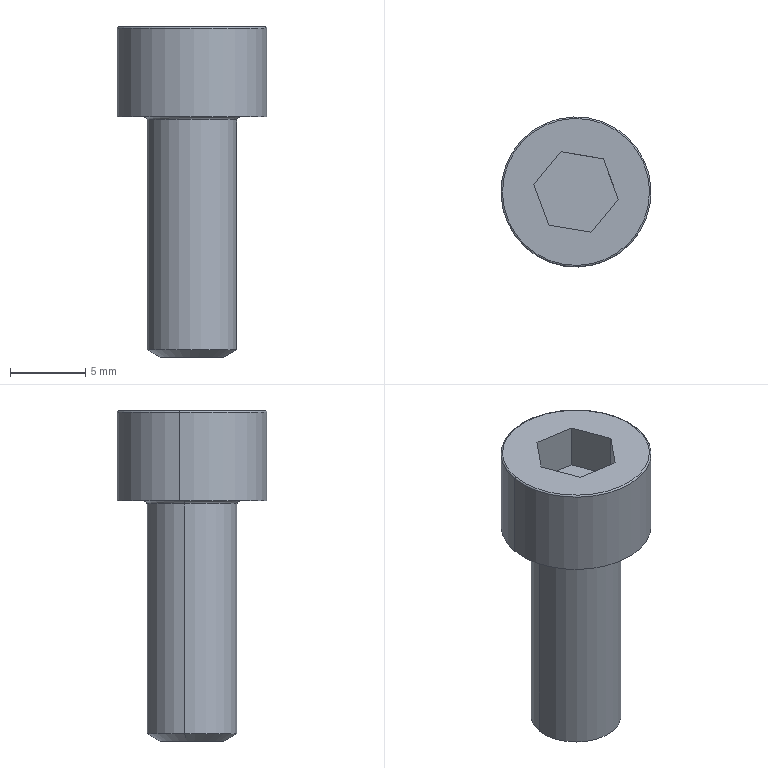Component | SolidWorks | GB_T70.1-2000_SocketHeadCapScrew_M6_16-1 | 1 solid | 20 faces | box 10 x 10 x 22 mm | volume 856 mm3 | plane 10 | torus 4 | cylinder 4 | cone 2 | commonest cylinder face diameters 10 x2 6 x2 | material 8.8 Grade
STEP:
#1=COLOUR_RGB('',0.7922,0.8196,0.9333);
#2=FILL_AREA_STYLE_COLOUR('',#1);
#3=FILL_AREA_STYLE('',(#2));
#4=SURFACE_STYLE_FILL_AREA(#3);
#5=SURFACE_SIDE_STYLE('',(#4));
#6=SURFACE_STYLE_USAGE(.BOTH.,#5);
#7=PRESENTATION_STYLE_ASSIGNMENT((#6));
#8=CARTESIAN_POINT('',(12.001,-2.129,19.252));
#9=VERTEX_POINT('',#8);
#10=CARTESIAN_POINT('',(11.621,-2.064,19.252));
#11=VERTEX_POINT('',#10);
#12=CARTESIAN_POINT('',(11.811,-2.096,19.252));
#13=DIRECTION('',(0.,-0.,1.));
#14=DIRECTION('',(-0.9861,0.1664,0.));
#15=AXIS2_PLACEMENT_3D('',#12,#13,#14);
#16=CIRCLE('',#15,0.1929);
#17=EDGE_CURVE('',#9,#11,#16,.T.);
#18=ORIENTED_EDGE('',*,*,#17,.F.);
#19=CARTESIAN_POINT('',(12.005,-2.129,19.248));
#20=VERTEX_POINT('',#19);
#21=CARTESIAN_POINT('',(12.001,-2.129,19.248));
#22=DIRECTION('',(0.1664,0.9861,-0.));
#23=DIRECTION('',(-0.9861,0.1664,0.));
#24=AXIS2_PLACEMENT_3D('',#21,#22,#23);
#25=CIRCLE('',#24,0.003937);
#26=EDGE_CURVE('',#9,#20,#25,.T.);
#27=ORIENTED_EDGE('',*,*,#26,.T.);
#28=CARTESIAN_POINT('',(11.617,-2.064,19.248));
#29=VERTEX_POINT('',#28);
#30=CARTESIAN_POINT('',(11.811,-2.096,19.248));
#31=DIRECTION('',(-0.,0.,-1.));
#32=DIRECTION('',(-0.9861,0.1664,0.));
#33=AXIS2_PLACEMENT_3D('',#30,#31,#32);
#34=CIRCLE('',#33,0.1969);
#35=EDGE_CURVE('',#29,#20,#34,.T.);
#36=ORIENTED_EDGE('',*,*,#35,.F.);
#37=CARTESIAN_POINT('',(11.621,-2.064,19.248));
#38=DIRECTION('',(-0.1664,-0.9861,0.));
#39=DIRECTION('',(0.9861,-0.1664,0.));
#40=AXIS2_PLACEMENT_3D('',#37,#38,#39);
#41=CIRCLE('',#40,0.003937);
#42=EDGE_CURVE('',#11,#29,#41,.T.);
#43=ORIENTED_EDGE('',*,*,#42,.F.);
#44=EDGE_LOOP('',(#18,#27,#36,#43));
#45=FACE_OUTER_BOUND('',#44,.T.);
#46=CARTESIAN_POINT('',(11.811,-2.096,19.248));
#47=DIRECTION('',(-0.,0.,-1.));
#48=DIRECTION('',(-0.9861,0.1664,0.));
#49=AXIS2_PLACEMENT_3D('',#46,#47,#48);
#50=TOROIDAL_SURFACE('',#49,0.1929,0.003937);
#51=ADVANCED_FACE('',(#45),#50,.T.);
#52=CARTESIAN_POINT('',(11.894,-2.11,18.386));
#53=VERTEX_POINT('',#52);
#54=CARTESIAN_POINT('',(11.728,-2.082,18.386));
#55=VERTEX_POINT('',#54);
#56=CARTESIAN_POINT('',(11.811,-2.096,18.386));
#57=DIRECTION('',(0.,-0.,1.));
#58=DIRECTION('',(0.9861,-0.1664,0.));
#59=AXIS2_PLACEMENT_3D('',#56,#57,#58);
#60=CIRCLE('',#59,0.08402);
#61=EDGE_CURVE('',#53,#55,#60,.T.);
#62=ORIENTED_EDGE('',*,*,#61,.T.);
#63=CARTESIAN_POINT('',(11.695,-2.077,18.406));
#64=VERTEX_POINT('',#63);
#65=CARTESIAN_POINT('',(11.695,-2.077,18.406));
#66=DIRECTION('',(-0.854,0.1441,0.5));
#67=VECTOR('',#66,39.37);
#68=LINE('',#65,#67);
#69=EDGE_CURVE('',#55,#64,#68,.T.);
#70=ORIENTED_EDGE('',*,*,#69,.T.);
#71=CARTESIAN_POINT('',(11.927,-2.116,18.406));
#72=VERTEX_POINT('',#71);
#73=CARTESIAN_POINT('',(11.811,-2.096,18.406));
#74=DIRECTION('',(0.,-0.,1.));
#75=DIRECTION('',(0.9861,-0.1664,0.));
#76=AXIS2_PLACEMENT_3D('',#73,#74,#75);
#77=CIRCLE('',#76,0.1181);
#78=EDGE_CURVE('',#72,#64,#77,.T.);
#79=ORIENTED_EDGE('',*,*,#78,.F.);
#80=CARTESIAN_POINT('',(11.927,-2.116,18.406));
#81=DIRECTION('',(0.854,-0.1441,0.5));
#82=VECTOR('',#81,39.37);
#83=LINE('',#80,#82);
#84=EDGE_CURVE('',#53,#72,#83,.T.);
#85=ORIENTED_EDGE('',*,*,#84,.F.);
#86=EDGE_LOOP('',(#62,#70,#79,#85));
#87=FACE_OUTER_BOUND('',#86,.T.);
#88=CARTESIAN_POINT('',(11.811,-2.096,18.406));
#89=DIRECTION('',(0.,-0.,1.));
#90=DIRECTION('',(0.9861,-0.1664,0.));
#91=AXIS2_PLACEMENT_3D('',#88,#89,#90);
#92=CONICAL_SURFACE('',#91,0.1181,1.047);
#93=ADVANCED_FACE('',(#87),#92,.T.);
#94=CARTESIAN_POINT('',(11.687,-2.075,19.016));
#95=VERTEX_POINT('',#94);
#96=CARTESIAN_POINT('',(11.935,-2.117,19.016));
#97=VERTEX_POINT('',#96);
#98=CARTESIAN_POINT('',(11.811,-2.096,19.016));
#99=DIRECTION('',(0.,-0.,1.));
#100=DIRECTION('',(0.9861,-0.1664,0.));
#101=AXIS2_PLACEMENT_3D('',#98,#99,#100);
#102=CIRCLE('',#101,0.126);
#103=EDGE_CURVE('',#95,#97,#102,.T.);
#104=ORIENTED_EDGE('',*,*,#103,.F.);
#105=CARTESIAN_POINT('',(11.695,-2.077,19.008));
#106=VERTEX_POINT('',#105);
#107=CARTESIAN_POINT('',(11.687,-2.075,19.008));
#108=DIRECTION('',(0.1664,0.9861,-0.));
#109=DIRECTION('',(-0.9861,0.1664,0.));
#110=AXIS2_PLACEMENT_3D('',#107,#108,#109);
#111=CIRCLE('',#110,0.007874);
#112=EDGE_CURVE('',#95,#106,#111,.T.);
#113=ORIENTED_EDGE('',*,*,#112,.T.);
#114=CARTESIAN_POINT('',(11.927,-2.116,19.008));
#115=VERTEX_POINT('',#114);
#116=CARTESIAN_POINT('',(11.811,-2.096,19.008));
#117=DIRECTION('',(0.,-0.,1.));
#118=DIRECTION('',(0.9861,-0.1664,0.));
#119=AXIS2_PLACEMENT_3D('',#116,#117,#118);
#120=CIRCLE('',#119,0.1181);
#121=EDGE_CURVE('',#106,#115,#120,.T.);
#122=ORIENTED_EDGE('',*,*,#121,.T.);
#123=CARTESIAN_POINT('',(11.935,-2.117,19.008));
#124=DIRECTION('',(-0.1664,-0.9861,0.));
#125=DIRECTION('',(0.9861,-0.1664,0.));
#126=AXIS2_PLACEMENT_3D('',#123,#124,#125);
#127=CIRCLE('',#126,0.007874);
#128=EDGE_CURVE('',#97,#115,#127,.T.);
#129=ORIENTED_EDGE('',*,*,#128,.F.);
#130=EDGE_LOOP('',(#104,#113,#122,#129));
#131=FACE_OUTER_BOUND('',#130,.T.);
#132=CARTESIAN_POINT('',(11.811,-2.096,19.008));
#133=DIRECTION('',(0.,-0.,1.));
#134=DIRECTION('',(0.9861,-0.1664,-0.));
#135=AXIS2_PLACEMENT_3D('',#132,#133,#134);
#136=TOROIDAL_SURFACE('',#135,0.126,0.007874);
#137=ADVANCED_FACE('',(#131),#136,.F.);
#138=CARTESIAN_POINT('',(12.005,-2.129,19.016));
#139=VERTEX_POINT('',#138);
#140=CARTESIAN_POINT('',(11.617,-2.064,19.016));
#141=VERTEX_POINT('',#140);
#142=CARTESIAN_POINT('',(11.811,-2.096,19.016));
#143=DIRECTION('',(0.,-0.,1.));
#144=DIRECTION('',(0.9861,-0.1664,0.));
#145=AXIS2_PLACEMENT_3D('',#142,#143,#144);
#146=CIRCLE('',#145,0.1969);
#147=EDGE_CURVE('',#139,#141,#146,.T.);
#148=ORIENTED_EDGE('',*,*,#147,.T.);
#149=CARTESIAN_POINT('',(11.617,-2.064,19.252));
#150=DIRECTION('',(0.,-0.,1.));
#151=VECTOR('',#150,39.37);
#152=LINE('',#149,#151);
#153=EDGE_CURVE('',#141,#29,#152,.T.);
#154=ORIENTED_EDGE('',*,*,#153,.T.);
#155=ORIENTED_EDGE('',*,*,#35,.T.);
#156=CARTESIAN_POINT('',(12.005,-2.129,19.252));
#157=DIRECTION('',(0.,-0.,1.));
#158=VECTOR('',#157,39.37);
#159=LINE('',#156,#158);
#160=EDGE_CURVE('',#139,#20,#159,.T.);
#161=ORIENTED_EDGE('',*,*,#160,.F.);
#162=EDGE_LOOP('',(#148,#154,#155,#161));
#163=FACE_OUTER_BOUND('',#162,.T.);
#164=CARTESIAN_POINT('',(11.811,-2.096,19.252));
#165=DIRECTION('',(0.,-0.,1.));
#166=DIRECTION('',(0.9861,-0.1664,0.));
#167=AXIS2_PLACEMENT_3D('',#164,#165,#166);
#168=CYLINDRICAL_SURFACE('',#167,0.1969);
#169=ADVANCED_FACE('',(#163),#168,.T.);
#170=ORIENTED_EDGE('',*,*,#78,.T.);
#171=CARTESIAN_POINT('',(11.695,-2.077,19.252));
#172=DIRECTION('',(0.,-0.,1.));
#173=VECTOR('',#172,39.37);
#174=LINE('',#171,#173);
#175=EDGE_CURVE('',#64,#106,#174,.T.);
#176=ORIENTED_EDGE('',*,*,#175,.T.);
#177=CARTESIAN_POINT('',(11.811,-2.096,19.008));
#178=DIRECTION('',(0.,-0.,1.));
#179=DIRECTION('',(0.9861,-0.1664,0.));
#180=AXIS2_PLACEMENT_3D('',#177,#178,#179);
#181=CIRCLE('',#180,0.1181);
#182=EDGE_CURVE('',#115,#106,#181,.T.);
#183=ORIENTED_EDGE('',*,*,#182,.F.);
#184=CARTESIAN_POINT('',(11.927,-2.116,19.252));
#185=DIRECTION('',(0.,-0.,1.));
#186=VECTOR('',#185,39.37);
#187=LINE('',#184,#186);
#188=EDGE_CURVE('',#72,#115,#187,.T.);
#189=ORIENTED_EDGE('',*,*,#188,.F.);
#190=EDGE_LOOP('',(#170,#176,#183,#189));
#191=FACE_OUTER_BOUND('',#190,.T.);
#192=CARTESIAN_POINT('',(11.811,-2.096,19.252));
#193=DIRECTION('',(0.,-0.,1.));
#194=DIRECTION('',(0.9861,-0.1664,0.));
#195=AXIS2_PLACEMENT_3D('',#192,#193,#194);
#196=CYLINDRICAL_SURFACE('',#195,0.1181);
#197=ADVANCED_FACE('',(#191),#196,.T.);
#198=ORIENTED_EDGE('',*,*,#175,.F.);
#199=CARTESIAN_POINT('',(11.811,-2.096,18.406));
#200=DIRECTION('',(0.,-0.,1.));
#201=DIRECTION('',(0.9861,-0.1664,0.));
#202=AXIS2_PLACEMENT_3D('',#199,#200,#201);
#203=CIRCLE('',#202,0.1181);
#204=EDGE_CURVE('',#64,#72,#203,.T.);
#205=ORIENTED_EDGE('',*,*,#204,.T.);
#206=ORIENTED_EDGE('',*,*,#188,.T.);
#207=ORIENTED_EDGE('',*,*,#121,.F.);
#208=EDGE_LOOP('',(#198,#205,#206,#207));
#209=FACE_OUTER_BOUND('',#208,.T.);
#210=CARTESIAN_POINT('',(11.811,-2.096,19.252));
#211=DIRECTION('',(0.,-0.,1.));
#212=DIRECTION('',(0.9861,-0.1664,0.));
#213=AXIS2_PLACEMENT_3D('',#210,#211,#212);
#214=CYLINDRICAL_SURFACE('',#213,0.1181);
#215=ADVANCED_FACE('',(#209),#214,.T.);
#216=CARTESIAN_POINT('',(11.811,-2.096,19.252));
#217=DIRECTION('',(0.,-0.,1.));
#218=DIRECTION('',(-0.9861,0.1664,0.));
#219=AXIS2_PLACEMENT_3D('',#216,#217,#218);
#220=CIRCLE('',#219,0.1929);
#221=EDGE_CURVE('',#11,#9,#220,.T.);
#222=ORIENTED_EDGE('',*,*,#221,.T.);
#223=ORIENTED_EDGE('',*,*,#17,.T.);
#224=EDGE_LOOP('',(#222,#223));
#225=FACE_OUTER_BOUND('',#224,.T.);
#226=CARTESIAN_POINT('',(11.922,-2.115,19.252));
#227=VERTEX_POINT('',#226);
#228=CARTESIAN_POINT('',(11.883,-2.01,19.252));
#229=VERTEX_POINT('',#228);
#230=CARTESIAN_POINT('',(11.922,-2.115,19.252));
#231=DIRECTION('',(-0.3489,0.9371,0.));
#232=VECTOR('',#231,39.37);
#233=LINE('',#230,#232);
#234=EDGE_CURVE('',#227,#229,#233,.T.);
#235=ORIENTED_EDGE('',*,*,#234,.F.);
#236=CARTESIAN_POINT('',(11.85,-2.202,19.252));
#237=VERTEX_POINT('',#236);
#238=CARTESIAN_POINT('',(11.85,-2.202,19.252));
#239=DIRECTION('',(0.6371,0.7708,-0.));
#240=VECTOR('',#239,39.37);
#241=LINE('',#238,#240);
#242=EDGE_CURVE('',#237,#227,#241,.T.);
#243=ORIENTED_EDGE('',*,*,#242,.F.);
#244=CARTESIAN_POINT('',(11.739,-2.183,19.252));
#245=VERTEX_POINT('',#244);
#246=CARTESIAN_POINT('',(11.739,-2.183,19.252));
#247=DIRECTION('',(0.9861,-0.1664,-0.));
#248=VECTOR('',#247,39.37);
#249=LINE('',#246,#248);
#250=EDGE_CURVE('',#245,#237,#249,.T.);
#251=ORIENTED_EDGE('',*,*,#250,.F.);
#252=CARTESIAN_POINT('',(11.7,-2.078,19.252));
#253=VERTEX_POINT('',#252);
#254=CARTESIAN_POINT('',(11.7,-2.078,19.252));
#255=DIRECTION('',(0.3489,-0.9371,-0.));
#256=VECTOR('',#255,39.37);
#257=LINE('',#254,#256);
#258=EDGE_CURVE('',#253,#245,#257,.T.);
#259=ORIENTED_EDGE('',*,*,#258,.F.);
#260=CARTESIAN_POINT('',(11.772,-1.991,19.252));
#261=VERTEX_POINT('',#260);
#262=CARTESIAN_POINT('',(11.772,-1.991,19.252));
#263=DIRECTION('',(-0.6371,-0.7708,0.));
#264=VECTOR('',#263,39.37);
#265=LINE('',#262,#264);
#266=EDGE_CURVE('',#261,#253,#265,.T.);
#267=ORIENTED_EDGE('',*,*,#266,.F.);
#268=CARTESIAN_POINT('',(11.883,-2.01,19.252));
#269=DIRECTION('',(-0.9861,0.1664,0.));
#270=VECTOR('',#269,39.37);
#271=LINE('',#268,#270);
#272=EDGE_CURVE('',#229,#261,#271,.T.);
#273=ORIENTED_EDGE('',*,*,#272,.F.);
#274=EDGE_LOOP('',(#235,#243,#251,#259,#267,#273));
#275=FACE_BOUND('',#274,.T.);
#276=CARTESIAN_POINT('',(11.811,-2.096,19.252));
#277=DIRECTION('',(-0.,0.,-1.));
#278=DIRECTION('',(-0.9861,0.1664,0.));
#279=AXIS2_PLACEMENT_3D('',#276,#277,#278);
#280=PLANE('',#279);
#281=ADVANCED_FACE('',(#225,#275),#280,.F.);
#282=ORIENTED_EDGE('',*,*,#153,.F.);
#283=CARTESIAN_POINT('',(11.811,-2.096,19.016));
#284=DIRECTION('',(0.,-0.,1.));
#285=DIRECTION('',(0.9861,-0.1664,0.));
#286=AXIS2_PLACEMENT_3D('',#283,#284,#285);
#287=CIRCLE('',#286,0.1969);
#288=EDGE_CURVE('',#141,#139,#287,.T.);
#289=ORIENTED_EDGE('',*,*,#288,.T.);
#290=ORIENTED_EDGE('',*,*,#160,.T.);
#291=CARTESIAN_POINT('',(11.811,-2.096,19.248));
#292=DIRECTION('',(-0.,0.,-1.));
#293=DIRECTION('',(-0.9861,0.1664,0.));
#294=AXIS2_PLACEMENT_3D('',#291,#292,#293);
#295=CIRCLE('',#294,0.1969);
#296=EDGE_CURVE('',#20,#29,#295,.T.);
#297=ORIENTED_EDGE('',*,*,#296,.T.);
#298=EDGE_LOOP('',(#282,#289,#290,#297));
#299=FACE_OUTER_BOUND('',#298,.T.);
#300=CARTESIAN_POINT('',(11.811,-2.096,19.252));
#301=DIRECTION('',(0.,-0.,1.));
#302=DIRECTION('',(0.9861,-0.1664,0.));
#303=AXIS2_PLACEMENT_3D('',#300,#301,#302);
#304=CYLINDRICAL_SURFACE('',#303,0.1969);
#305=ADVANCED_FACE('',(#299),#304,.T.);
#306=ORIENTED_EDGE('',*,*,#147,.F.);
#307=ORIENTED_EDGE('',*,*,#288,.F.);
#308=EDGE_LOOP('',(#306,#307));
#309=FACE_OUTER_BOUND('',#308,.T.);
#310=CARTESIAN_POINT('',(11.811,-2.096,19.016));
#311=DIRECTION('',(0.,-0.,1.));
#312=DIRECTION('',(0.9861,-0.1664,0.));
#313=AXIS2_PLACEMENT_3D('',#310,#311,#312);
#314=CIRCLE('',#313,0.126);
#315=EDGE_CURVE('',#97,#95,#314,.T.);
#316=ORIENTED_EDGE('',*,*,#315,.T.);
#317=ORIENTED_EDGE('',*,*,#103,.T.);
#318=EDGE_LOOP('',(#316,#317));
#319=FACE_BOUND('',#318,.T.);
#320=CARTESIAN_POINT('',(11.844,-1.902,19.016));
#321=DIRECTION('',(0.,-0.,1.));
#322=DIRECTION('',(0.9861,-0.1664,-0.));
#323=AXIS2_PLACEMENT_3D('',#320,#321,#322);
#324=PLANE('',#323);
#325=ADVANCED_FACE('',(#309,#319),#324,.F.);
#326=ORIENTED_EDGE('',*,*,#112,.F.);
#327=ORIENTED_EDGE('',*,*,#315,.F.);
#328=ORIENTED_EDGE('',*,*,#128,.T.);
#329=ORIENTED_EDGE('',*,*,#182,.T.);
#330=EDGE_LOOP('',(#326,#327,#328,#329));
#331=FACE_OUTER_BOUND('',#330,.T.);
#332=CARTESIAN_POINT('',(11.811,-2.096,19.008));
#333=DIRECTION('',(0.,-0.,1.));
#334=DIRECTION('',(0.9861,-0.1664,-0.));
#335=AXIS2_PLACEMENT_3D('',#332,#333,#334);
#336=TOROIDAL_SURFACE('',#335,0.126,0.007874);
#337=ADVANCED_FACE('',(#331),#336,.F.);
#338=ORIENTED_EDGE('',*,*,#242,.T.);
#339=CARTESIAN_POINT('',(11.922,-2.115,19.134));
#340=VERTEX_POINT('',#339);
#341=CARTESIAN_POINT('',(11.922,-2.115,19.134));
#342=DIRECTION('',(0.,-0.,1.));
#343=VECTOR('',#342,39.37);
#344=LINE('',#341,#343);
#345=EDGE_CURVE('',#340,#227,#344,.T.);
#346=ORIENTED_EDGE('',*,*,#345,.F.);
#347=CARTESIAN_POINT('',(11.85,-2.202,19.134));
#348=VERTEX_POINT('',#347);
#349=CARTESIAN_POINT('',(11.85,-2.202,19.134));
#350=DIRECTION('',(0.6371,0.7708,-0.));
#351=VECTOR('',#350,39.37);
#352=LINE('',#349,#351);
#353=EDGE_CURVE('',#348,#340,#352,.T.);
#354=ORIENTED_EDGE('',*,*,#353,.F.);
#355=CARTESIAN_POINT('',(11.85,-2.202,19.134));
#356=DIRECTION('',(0.,-0.,1.));
#357=VECTOR('',#356,39.37);
#358=LINE('',#355,#357);
#359=EDGE_CURVE('',#348,#237,#358,.T.);
#360=ORIENTED_EDGE('',*,*,#359,.T.);
#361=EDGE_LOOP('',(#338,#346,#354,#360));
#362=FACE_OUTER_BOUND('',#361,.T.);
#363=CARTESIAN_POINT('',(11.85,-2.202,19.134));
#364=DIRECTION('',(0.7708,-0.6371,-0.));
#365=DIRECTION('',(-0.6371,-0.7708,0.));
#366=AXIS2_PLACEMENT_3D('',#363,#364,#365);
#367=PLANE('',#366);
#368=ADVANCED_FACE('',(#362),#367,.F.);
#369=ORIENTED_EDGE('',*,*,#250,.T.);
#370=ORIENTED_EDGE('',*,*,#359,.F.);
#371=CARTESIAN_POINT('',(11.739,-2.183,19.134));
#372=VERTEX_POINT('',#371);
#373=CARTESIAN_POINT('',(11.739,-2.183,19.134));
#374=DIRECTION('',(0.9861,-0.1664,-0.));
#375=VECTOR('',#374,39.37);
#376=LINE('',#373,#375);
#377=EDGE_CURVE('',#372,#348,#376,.T.);
#378=ORIENTED_EDGE('',*,*,#377,.F.);
#379=CARTESIAN_POINT('',(11.739,-2.183,19.134));
#380=DIRECTION('',(0.,-0.,1.));
#381=VECTOR('',#380,39.37);
#382=LINE('',#379,#381);
#383=EDGE_CURVE('',#372,#245,#382,.T.);
#384=ORIENTED_EDGE('',*,*,#383,.T.);
#385=EDGE_LOOP('',(#369,#370,#378,#384));
#386=FACE_OUTER_BOUND('',#385,.T.);
#387=CARTESIAN_POINT('',(11.739,-2.183,19.134));
#388=DIRECTION('',(-0.1664,-0.9861,0.));
#389=DIRECTION('',(-0.9861,0.1664,0.));
#390=AXIS2_PLACEMENT_3D('',#387,#388,#389);
#391=PLANE('',#390);
#392=ADVANCED_FACE('',(#386),#391,.F.);
#393=ORIENTED_EDGE('',*,*,#258,.T.);
#394=ORIENTED_EDGE('',*,*,#383,.F.);
#395=CARTESIAN_POINT('',(11.7,-2.078,19.134));
#396=VERTEX_POINT('',#395);
#397=CARTESIAN_POINT('',(11.7,-2.078,19.134));
#398=DIRECTION('',(0.3489,-0.9371,-0.));
#399=VECTOR('',#398,39.37);
#400=LINE('',#397,#399);
#401=EDGE_CURVE('',#396,#372,#400,.T.);
#402=ORIENTED_EDGE('',*,*,#401,.F.);
#403=CARTESIAN_POINT('',(11.7,-2.078,19.134));
#404=DIRECTION('',(0.,-0.,1.));
#405=VECTOR('',#404,39.37);
#406=LINE('',#403,#405);
#407=EDGE_CURVE('',#396,#253,#406,.T.);
#408=ORIENTED_EDGE('',*,*,#407,.T.);
#409=EDGE_LOOP('',(#393,#394,#402,#408));
#410=FACE_OUTER_BOUND('',#409,.T.);
#411=CARTESIAN_POINT('',(11.7,-2.078,19.134));
#412=DIRECTION('',(-0.9371,-0.3489,0.));
#413=DIRECTION('',(-0.3489,0.9371,0.));
#414=AXIS2_PLACEMENT_3D('',#411,#412,#413);
#415=PLANE('',#414);
#416=ADVANCED_FACE('',(#410),#415,.F.);
#417=ORIENTED_EDGE('',*,*,#266,.T.);
#418=ORIENTED_EDGE('',*,*,#407,.F.);
#419=CARTESIAN_POINT('',(11.772,-1.991,19.134));
#420=VERTEX_POINT('',#419);
#421=CARTESIAN_POINT('',(11.772,-1.991,19.134));
#422=DIRECTION('',(-0.6371,-0.7708,0.));
#423=VECTOR('',#422,39.37);
#424=LINE('',#421,#423);
#425=EDGE_CURVE('',#420,#396,#424,.T.);
#426=ORIENTED_EDGE('',*,*,#425,.F.);
#427=CARTESIAN_POINT('',(11.772,-1.991,19.134));
#428=DIRECTION('',(0.,-0.,1.));
#429=VECTOR('',#428,39.37);
#430=LINE('',#427,#429);
#431=EDGE_CURVE('',#420,#261,#430,.T.);
#432=ORIENTED_EDGE('',*,*,#431,.T.);
#433=EDGE_LOOP('',(#417,#418,#426,#432));
#434=FACE_OUTER_BOUND('',#433,.T.);
#435=CARTESIAN_POINT('',(11.772,-1.991,19.134));
#436=DIRECTION('',(-0.7708,0.6371,0.));
#437=DIRECTION('',(0.6371,0.7708,-0.));
#438=AXIS2_PLACEMENT_3D('',#435,#436,#437);
#439=PLANE('',#438);
#440=ADVANCED_FACE('',(#434),#439,.F.);
#441=ORIENTED_EDGE('',*,*,#272,.T.);
#442=ORIENTED_EDGE('',*,*,#431,.F.);
#443=CARTESIAN_POINT('',(11.883,-2.01,19.134));
#444=VERTEX_POINT('',#443);
#445=CARTESIAN_POINT('',(11.883,-2.01,19.134));
#446=DIRECTION('',(-0.9861,0.1664,0.));
#447=VECTOR('',#446,39.37);
#448=LINE('',#445,#447);
#449=EDGE_CURVE('',#444,#420,#448,.T.);
#450=ORIENTED_EDGE('',*,*,#449,.F.);
#451=CARTESIAN_POINT('',(11.883,-2.01,19.134));
#452=DIRECTION('',(0.,-0.,1.));
#453=VECTOR('',#452,39.37);
#454=LINE('',#451,#453);
#455=EDGE_CURVE('',#444,#229,#454,.T.);
#456=ORIENTED_EDGE('',*,*,#455,.T.);
#457=EDGE_LOOP('',(#441,#442,#450,#456));
#458=FACE_OUTER_BOUND('',#457,.T.);
#459=CARTESIAN_POINT('',(11.883,-2.01,19.134));
#460=DIRECTION('',(0.1664,0.9861,-0.));
#461=DIRECTION('',(0.9861,-0.1664,-0.));
#462=AXIS2_PLACEMENT_3D('',#459,#460,#461);
#463=PLANE('',#462);
#464=ADVANCED_FACE('',(#458),#463,.F.);
#465=ORIENTED_EDGE('',*,*,#234,.T.);
#466=ORIENTED_EDGE('',*,*,#455,.F.);
#467=CARTESIAN_POINT('',(11.922,-2.115,19.134));
#468=DIRECTION('',(-0.3489,0.9371,0.));
#469=VECTOR('',#468,39.37);
#470=LINE('',#467,#469);
#471=EDGE_CURVE('',#340,#444,#470,.T.);
#472=ORIENTED_EDGE('',*,*,#471,.F.);
#473=ORIENTED_EDGE('',*,*,#345,.T.);
#474=EDGE_LOOP('',(#465,#466,#472,#473));
#475=FACE_OUTER_BOUND('',#474,.T.);
#476=CARTESIAN_POINT('',(11.922,-2.115,19.134));
#477=DIRECTION('',(0.9371,0.3489,-0.));
#478=DIRECTION('',(0.3489,-0.9371,-0.));
#479=AXIS2_PLACEMENT_3D('',#476,#477,#478);
#480=PLANE('',#479);
#481=ADVANCED_FACE('',(#475),#480,.F.);
#482=ORIENTED_EDGE('',*,*,#353,.T.);
#483=ORIENTED_EDGE('',*,*,#471,.T.);
#484=ORIENTED_EDGE('',*,*,#449,.T.);
#485=ORIENTED_EDGE('',*,*,#425,.T.);
#486=ORIENTED_EDGE('',*,*,#401,.T.);
#487=ORIENTED_EDGE('',*,*,#377,.T.);
#488=EDGE_LOOP('',(#482,#483,#484,#485,#486,#487));
#489=FACE_OUTER_BOUND('',#488,.T.);
#490=CARTESIAN_POINT('',(11.85,-2.202,19.134));
#491=DIRECTION('',(-0.,0.,-1.));
#492=DIRECTION('',(-0.9861,0.1664,0.));
#493=AXIS2_PLACEMENT_3D('',#490,#491,#492);
#494=PLANE('',#493);
#495=ADVANCED_FACE('',(#489),#494,.F.);
#496=ORIENTED_EDGE('',*,*,#69,.F.);
#497=CARTESIAN_POINT('',(11.811,-2.096,18.386));
#498=DIRECTION('',(0.,-0.,1.));
#499=DIRECTION('',(0.9861,-0.1664,0.));
#500=AXIS2_PLACEMENT_3D('',#497,#498,#499);
#501=CIRCLE('',#500,0.08402);
#502=EDGE_CURVE('',#55,#53,#501,.T.);
#503=ORIENTED_EDGE('',*,*,#502,.T.);
#504=ORIENTED_EDGE('',*,*,#84,.T.);
#505=ORIENTED_EDGE('',*,*,#204,.F.);
#506=EDGE_LOOP('',(#496,#503,#504,#505));
#507=FACE_OUTER_BOUND('',#506,.T.);
#508=CARTESIAN_POINT('',(11.811,-2.096,18.406));
#509=DIRECTION('',(0.,-0.,1.));
#510=DIRECTION('',(0.9861,-0.1664,0.));
#511=AXIS2_PLACEMENT_3D('',#508,#509,#510);
#512=CONICAL_SURFACE('',#511,0.1181,1.047);
#513=ADVANCED_FACE('',(#507),#512,.T.);
#514=ORIENTED_EDGE('',*,*,#61,.F.);
#515=ORIENTED_EDGE('',*,*,#502,.F.);
#516=EDGE_LOOP('',(#514,#515));
#517=FACE_OUTER_BOUND('',#516,.T.);
#518=CARTESIAN_POINT('',(11.831,-1.98,18.386));
#519=DIRECTION('',(0.,-0.,1.));
#520=DIRECTION('',(0.9861,-0.1664,-0.));
#521=AXIS2_PLACEMENT_3D('',#518,#519,#520);
#522=PLANE('',#521);
#523=ADVANCED_FACE('',(#517),#522,.F.);
#524=ORIENTED_EDGE('',*,*,#26,.F.);
#525=ORIENTED_EDGE('',*,*,#221,.F.);
#526=ORIENTED_EDGE('',*,*,#42,.T.);
#527=ORIENTED_EDGE('',*,*,#296,.F.);
#528=EDGE_LOOP('',(#524,#525,#526,#527));
#529=FACE_OUTER_BOUND('',#528,.T.);
#530=CARTESIAN_POINT('',(11.811,-2.096,19.248));
#531=DIRECTION('',(-0.,0.,-1.));
#532=DIRECTION('',(-0.9861,0.1664,0.));
#533=AXIS2_PLACEMENT_3D('',#530,#531,#532);
#534=TOROIDAL_SURFACE('',#533,0.1929,0.003937);
#535=ADVANCED_FACE('',(#529),#534,.T.);
#536=CLOSED_SHELL('',(#51,#93,#137,#169,#197,#215,#281,#305,#325,#337,#368,#392,#416,#440,#464,#481,#495,#513,#523,#535));
#537=MANIFOLD_SOLID_BREP('',#536);
#538=STYLED_ITEM('',(#7),#537);
#539=(LENGTH_UNIT()NAMED_UNIT(*)SI_UNIT($,.METRE.));
#540=LENGTH_MEASURE_WITH_UNIT(LENGTH_MEASURE(0.0254),#539);
#541=DIMENSIONAL_EXPONENTS(1.,0.,0.,0.,0.,0.,0.);
#542=(CONVERSION_BASED_UNIT('',#540)LENGTH_UNIT()NAMED_UNIT(#541));
#543=UNCERTAINTY_MEASURE_WITH_UNIT(LENGTH_MEASURE(0.00001),#542,'','');
#544=(NAMED_UNIT(*)PLANE_ANGLE_UNIT()SI_UNIT($,.RADIAN.));
#545=(NAMED_UNIT(*)SI_UNIT($,.STERADIAN.)SOLID_ANGLE_UNIT());
#546=(GEOMETRIC_REPRESENTATION_CONTEXT(3)GLOBAL_UNCERTAINTY_ASSIGNED_CONTEXT((#543))GLOBAL_UNIT_ASSIGNED_CONTEXT((#542,#544,#545))REPRESENTATION_CONTEXT('',''));
#547=MECHANICAL_DESIGN_GEOMETRIC_PRESENTATION_REPRESENTATION('',(#538),#546);
#548=CARTESIAN_POINT('',(0.,0.,0.));
#549=DIRECTION('',(0.,0.,1.));
#550=DIRECTION('',(1.,0.,0.));
#551=AXIS2_PLACEMENT_3D('',#548,#549,#550);
#552=(LENGTH_UNIT()NAMED_UNIT(*)SI_UNIT($,.METRE.));
#553=LENGTH_MEASURE_WITH_UNIT(LENGTH_MEASURE(0.0254),#552);
#554=DIMENSIONAL_EXPONENTS(1.,0.,0.,0.,0.,0.,0.);
#555=(CONVERSION_BASED_UNIT('',#553)LENGTH_UNIT()NAMED_UNIT(#554));
#556=UNCERTAINTY_MEASURE_WITH_UNIT(LENGTH_MEASURE(0.00001),#555,'','');
#557=(NAMED_UNIT(*)PLANE_ANGLE_UNIT()SI_UNIT($,.RADIAN.));
#558=(NAMED_UNIT(*)SI_UNIT($,.STERADIAN.)SOLID_ANGLE_UNIT());
#559=(GEOMETRIC_REPRESENTATION_CONTEXT(3)GLOBAL_UNCERTAINTY_ASSIGNED_CONTEXT((#556))GLOBAL_UNIT_ASSIGNED_CONTEXT((#555,#557,#558))REPRESENTATION_CONTEXT('',''));
#560=ADVANCED_BREP_SHAPE_REPRESENTATION('',(#537,#551),#559);
#561=PRESENTATION_LAYER_ASSIGNMENT('','',(#538));